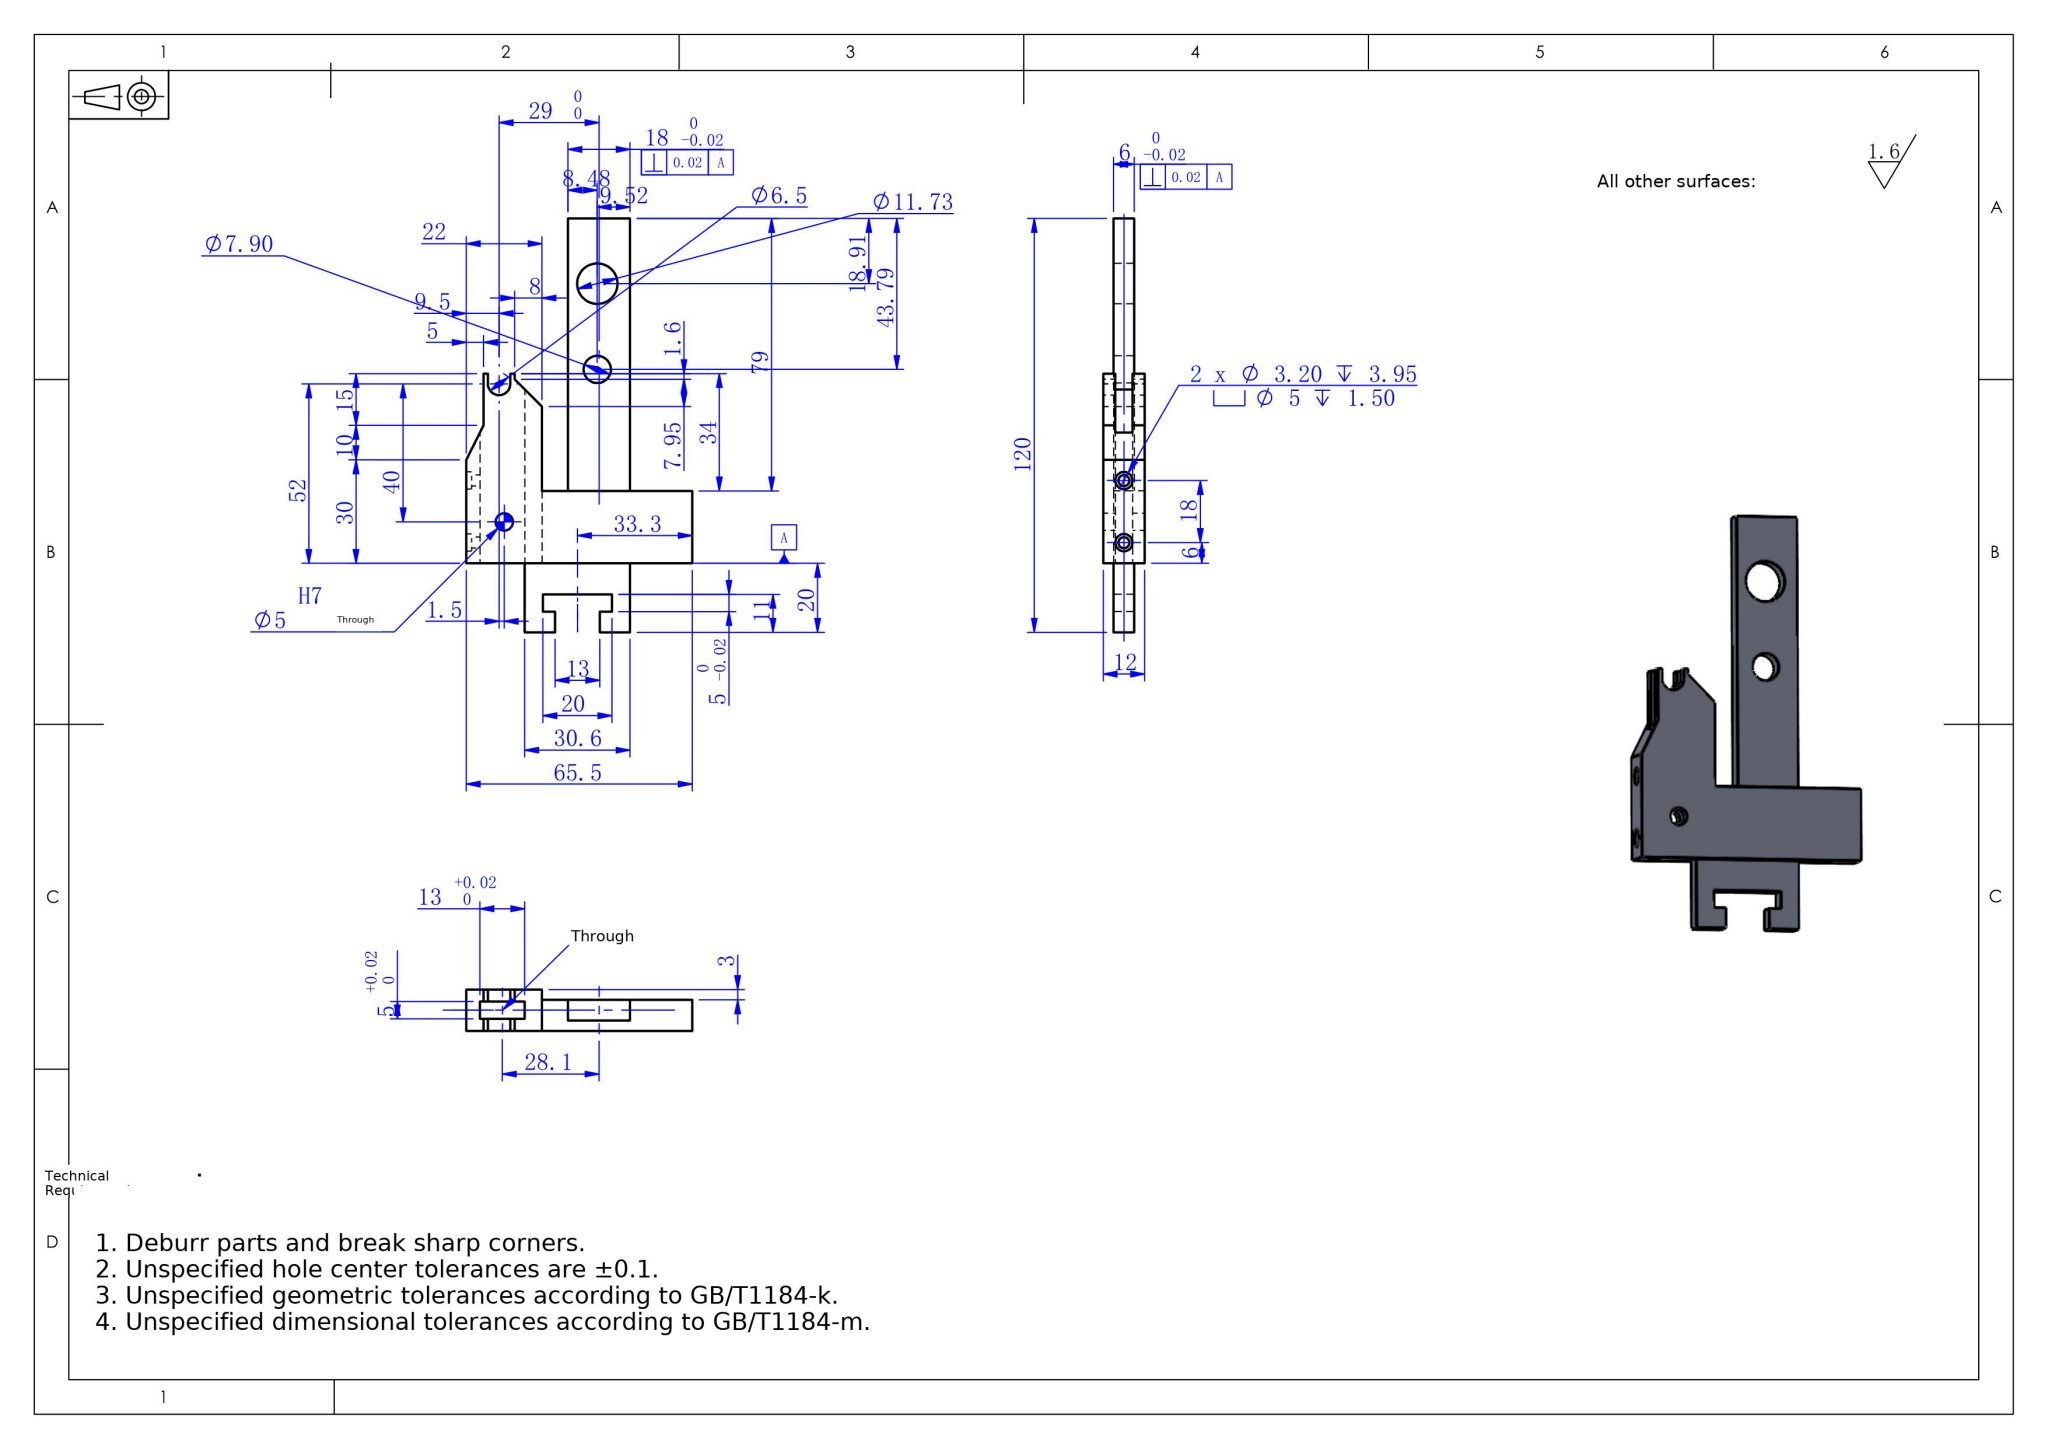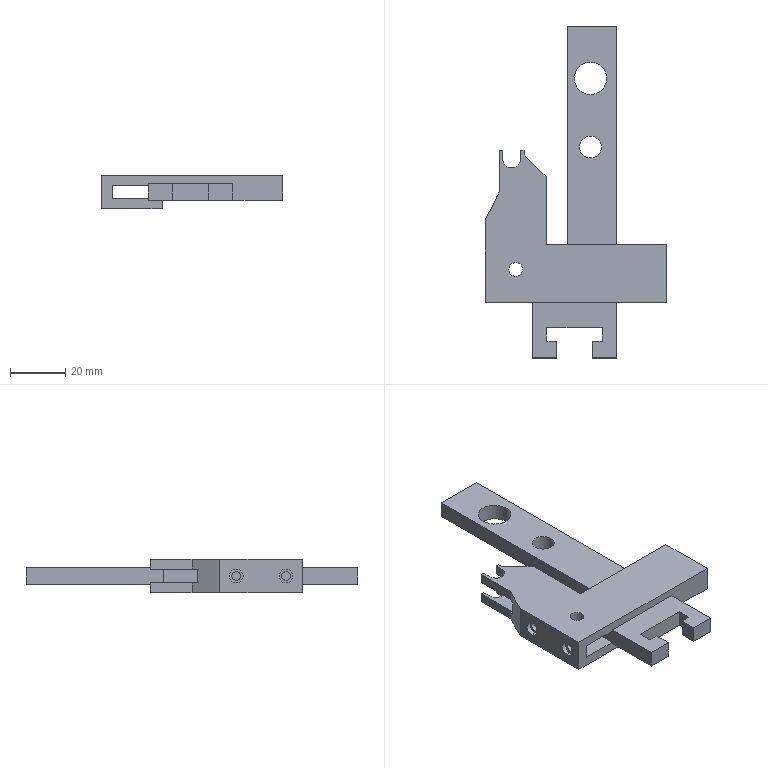Part | SolidWorks | mm | 1 solid | 61 faces | box 65.5 x 120 x 12 mm | volume 27239 mm3 | plane 43 | cylinder 18 | commonest cylinder face diameters 5 x8 3.2 x4 11.727 x2 7.904 x2 6.5 x2